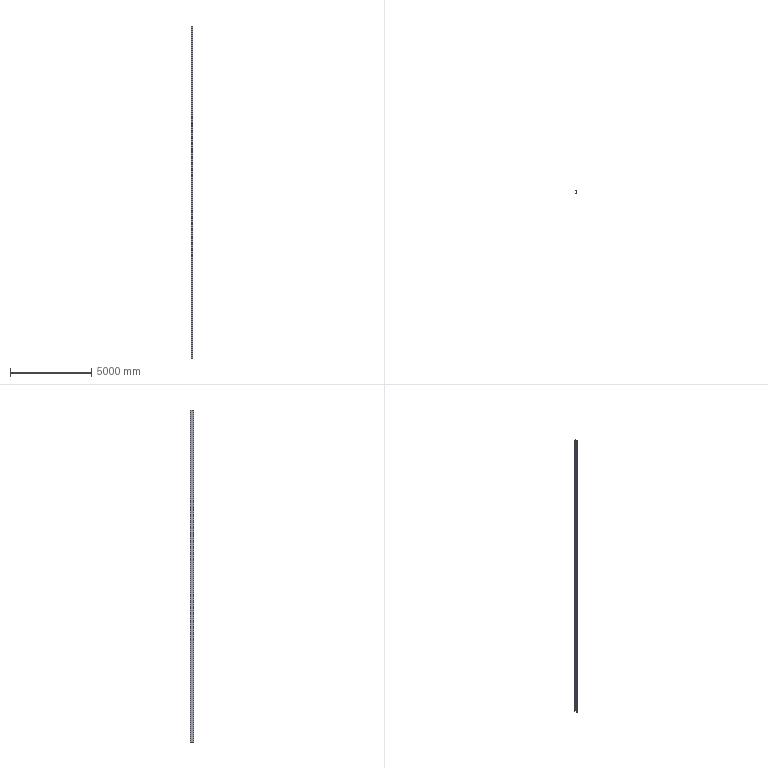Component | NX | P3 | 1 solid | 12 faces | box 73 x 200 x 20380 mm | volume 59182168 mm3 | plane 10 | cylinder 2 | commonest cylinder face diameters 22 x2
STEP:
#1=CARTESIAN_POINT('',(0.,0.,0.));
#2=DIRECTION('',(0.,0.,1.));
#3=DIRECTION('',(1.,0.,0.));
#4=AXIS2_PLACEMENT_3D('',#1,#2,#3);
#5=CARTESIAN_POINT('',(6830.,-6.,4.));
#6=VERTEX_POINT('',#5);
#7=CARTESIAN_POINT('',(6757.,-6.,4.));
#8=VERTEX_POINT('',#7);
#9=CARTESIAN_POINT('',(6830.,-6.,4.));
#10=DIRECTION('',(-1.,-0.,0.));
#11=VECTOR('',#10,1.);
#12=LINE('',#9,#11);
#13=CARTESIAN_POINT('',(6830.,-6.,20384.));
#14=DIRECTION('',(0.,-1.,0.));
#15=DIRECTION('',(-1.,-0.,0.));
#16=AXIS2_PLACEMENT_3D('',#13,#14,#15);
#17=PLANE('',#16);
#18=CARTESIAN_POINT('',(0.,20380.));
#19=DIRECTION('',(1.,0.));
#20=VECTOR('',#19,1.);
#21=LINE('',#18,#20);
#22=(GEOMETRIC_REPRESENTATION_CONTEXT(2)PARAMETRIC_REPRESENTATION_CONTEXT()REPRESENTATION_CONTEXT('',''));
#23=DEFINITIONAL_REPRESENTATION('',(#21),#22);
#24=PCURVE('',#17,#23);
#25=CARTESIAN_POINT('',(6812.,-28.,4.));
#26=DIRECTION('',(0.,0.,-1.));
#27=DIRECTION('',(0.,-1.,0.));
#28=AXIS2_PLACEMENT_3D('',#25,#26,#27);
#29=PLANE('',#28);
#30=CARTESIAN_POINT('',(-22.,-18.));
#31=DIRECTION('',(0.,1.));
#32=VECTOR('',#31,1.);
#33=LINE('',#30,#32);
#34=(GEOMETRIC_REPRESENTATION_CONTEXT(2)PARAMETRIC_REPRESENTATION_CONTEXT()REPRESENTATION_CONTEXT('',''));
#35=DEFINITIONAL_REPRESENTATION('',(#33),#34);
#36=PCURVE('',#29,#35);
#37=SURFACE_CURVE('',#12,(#24,#36),.PCURVE_S1.);
#38=EDGE_CURVE('',#6,#8,#37,.T.);
#39=ORIENTED_EDGE('',*,*,#38,.T.);
#40=CARTESIAN_POINT('',(6757.,-6.,20384.));
#41=VERTEX_POINT('',#40);
#42=CARTESIAN_POINT('',(6757.,-6.,20384.));
#43=DIRECTION('',(0.,0.,-1.));
#44=VECTOR('',#43,1.);
#45=LINE('',#42,#44);
#46=CARTESIAN_POINT('',(73.,0.));
#47=DIRECTION('',(0.,1.));
#48=VECTOR('',#47,1.);
#49=LINE('',#46,#48);
#50=(GEOMETRIC_REPRESENTATION_CONTEXT(2)PARAMETRIC_REPRESENTATION_CONTEXT()REPRESENTATION_CONTEXT('',''));
#51=DEFINITIONAL_REPRESENTATION('',(#49),#50);
#52=PCURVE('',#17,#51);
#53=CARTESIAN_POINT('',(6757.,-6.,20384.));
#54=DIRECTION('',(1.,0.,0.));
#55=DIRECTION('',(0.,0.,1.));
#56=AXIS2_PLACEMENT_3D('',#53,#54,#55);
#57=PLANE('',#56);
#58=CARTESIAN_POINT('',(0.,0.));
#59=DIRECTION('',(-1.,0.));
#60=VECTOR('',#59,1.);
#61=LINE('',#58,#60);
#62=(GEOMETRIC_REPRESENTATION_CONTEXT(2)PARAMETRIC_REPRESENTATION_CONTEXT()REPRESENTATION_CONTEXT('',''));
#63=DEFINITIONAL_REPRESENTATION('',(#61),#62);
#64=PCURVE('',#57,#63);
#65=SURFACE_CURVE('',#45,(#52,#64),.PCURVE_S1.);
#66=EDGE_CURVE('',#41,#8,#65,.T.);
#67=ORIENTED_EDGE('',*,*,#66,.F.);
#68=CARTESIAN_POINT('',(6830.,-6.,20384.));
#69=VERTEX_POINT('',#68);
#70=CARTESIAN_POINT('',(6830.,-6.,20384.));
#71=DIRECTION('',(-1.,-0.,0.));
#72=VECTOR('',#71,1.);
#73=LINE('',#70,#72);
#74=CARTESIAN_POINT('',(0.,0.));
#75=DIRECTION('',(1.,0.));
#76=VECTOR('',#75,1.);
#77=LINE('',#74,#76);
#78=(GEOMETRIC_REPRESENTATION_CONTEXT(2)PARAMETRIC_REPRESENTATION_CONTEXT()REPRESENTATION_CONTEXT('',''));
#79=DEFINITIONAL_REPRESENTATION('',(#77),#78);
#80=PCURVE('',#17,#79);
#81=CARTESIAN_POINT('',(6812.,-28.,20384.));
#82=DIRECTION('',(0.,0.,-1.));
#83=DIRECTION('',(0.,-1.,0.));
#84=AXIS2_PLACEMENT_3D('',#81,#82,#83);
#85=PLANE('',#84);
#86=CARTESIAN_POINT('',(-22.,-18.));
#87=DIRECTION('',(0.,1.));
#88=VECTOR('',#87,1.);
#89=LINE('',#86,#88);
#90=(GEOMETRIC_REPRESENTATION_CONTEXT(2)PARAMETRIC_REPRESENTATION_CONTEXT()REPRESENTATION_CONTEXT('',''));
#91=DEFINITIONAL_REPRESENTATION('',(#89),#90);
#92=PCURVE('',#85,#91);
#93=SURFACE_CURVE('',#73,(#80,#92),.PCURVE_S1.);
#94=EDGE_CURVE('',#69,#41,#93,.T.);
#95=ORIENTED_EDGE('',*,*,#94,.F.);
#96=CARTESIAN_POINT('',(6830.,-6.,20384.));
#97=DIRECTION('',(0.,0.,-1.));
#98=VECTOR('',#97,1.);
#99=LINE('',#96,#98);
#100=CARTESIAN_POINT('',(0.,0.));
#101=DIRECTION('',(0.,1.));
#102=VECTOR('',#101,1.);
#103=LINE('',#100,#102);
#104=(GEOMETRIC_REPRESENTATION_CONTEXT(2)PARAMETRIC_REPRESENTATION_CONTEXT()REPRESENTATION_CONTEXT('',''));
#105=DEFINITIONAL_REPRESENTATION('',(#103),#104);
#106=PCURVE('',#17,#105);
#107=CARTESIAN_POINT('',(6830.,-206.,20384.));
#108=DIRECTION('',(-1.,0.,0.));
#109=DIRECTION('',(0.,0.,-1.));
#110=AXIS2_PLACEMENT_3D('',#107,#108,#109);
#111=PLANE('',#110);
#112=CARTESIAN_POINT('',(0.,-200.));
#113=DIRECTION('',(1.,0.));
#114=VECTOR('',#113,1.);
#115=LINE('',#112,#114);
#116=(GEOMETRIC_REPRESENTATION_CONTEXT(2)PARAMETRIC_REPRESENTATION_CONTEXT()REPRESENTATION_CONTEXT('',''));
#117=DEFINITIONAL_REPRESENTATION('',(#115),#116);
#118=PCURVE('',#111,#117);
#119=SURFACE_CURVE('',#99,(#106,#118),.PCURVE_S1.);
#120=EDGE_CURVE('',#69,#6,#119,.T.);
#121=ORIENTED_EDGE('',*,*,#120,.T.);
#122=EDGE_LOOP('',(#39,#67,#95,#121));
#123=FACE_BOUND('',#122,.T.);
#124=ADVANCED_FACE('',(#123),#17,.F.);
#125=CARTESIAN_POINT('',(6757.,-17.,4.));
#126=VERTEX_POINT('',#125);
#127=CARTESIAN_POINT('',(6757.,-6.,4.));
#128=DIRECTION('',(0.,-1.,0.));
#129=VECTOR('',#128,1.);
#130=LINE('',#127,#129);
#131=CARTESIAN_POINT('',(-20380.,0.));
#132=DIRECTION('',(0.,1.));
#133=VECTOR('',#132,1.);
#134=LINE('',#131,#133);
#135=(GEOMETRIC_REPRESENTATION_CONTEXT(2)PARAMETRIC_REPRESENTATION_CONTEXT()REPRESENTATION_CONTEXT('',''));
#136=DEFINITIONAL_REPRESENTATION('',(#134),#135);
#137=PCURVE('',#57,#136);
#138=CARTESIAN_POINT('',(-22.,55.));
#139=DIRECTION('',(1.,0.));
#140=VECTOR('',#139,1.);
#141=LINE('',#138,#140);
#142=(GEOMETRIC_REPRESENTATION_CONTEXT(2)PARAMETRIC_REPRESENTATION_CONTEXT()REPRESENTATION_CONTEXT('',''));
#143=DEFINITIONAL_REPRESENTATION('',(#141),#142);
#144=PCURVE('',#29,#143);
#145=SURFACE_CURVE('',#130,(#137,#144),.PCURVE_S1.);
#146=EDGE_CURVE('',#8,#126,#145,.T.);
#147=ORIENTED_EDGE('',*,*,#146,.T.);
#148=CARTESIAN_POINT('',(6757.,-17.,20384.));
#149=VERTEX_POINT('',#148);
#150=CARTESIAN_POINT('',(6757.,-17.,20384.));
#151=DIRECTION('',(0.,0.,-1.));
#152=VECTOR('',#151,1.);
#153=LINE('',#150,#152);
#154=CARTESIAN_POINT('',(0.,11.));
#155=DIRECTION('',(-1.,0.));
#156=VECTOR('',#155,1.);
#157=LINE('',#154,#156);
#158=(GEOMETRIC_REPRESENTATION_CONTEXT(2)PARAMETRIC_REPRESENTATION_CONTEXT()REPRESENTATION_CONTEXT('',''));
#159=DEFINITIONAL_REPRESENTATION('',(#157),#158);
#160=PCURVE('',#57,#159);
#161=CARTESIAN_POINT('',(6757.,-17.,20384.));
#162=DIRECTION('',(-0.,1.,0.));
#163=DIRECTION('',(1.,0.,0.));
#164=AXIS2_PLACEMENT_3D('',#161,#162,#163);
#165=PLANE('',#164);
#166=CARTESIAN_POINT('',(0.,0.));
#167=DIRECTION('',(0.,1.));
#168=VECTOR('',#167,1.);
#169=LINE('',#166,#168);
#170=(GEOMETRIC_REPRESENTATION_CONTEXT(2)PARAMETRIC_REPRESENTATION_CONTEXT()REPRESENTATION_CONTEXT('',''));
#171=DEFINITIONAL_REPRESENTATION('',(#169),#170);
#172=PCURVE('',#165,#171);
#173=SURFACE_CURVE('',#153,(#160,#172),.PCURVE_S1.);
#174=EDGE_CURVE('',#149,#126,#173,.T.);
#175=ORIENTED_EDGE('',*,*,#174,.F.);
#176=CARTESIAN_POINT('',(6757.,-6.,20384.));
#177=DIRECTION('',(0.,-1.,0.));
#178=VECTOR('',#177,1.);
#179=LINE('',#176,#178);
#180=CARTESIAN_POINT('',(0.,0.));
#181=DIRECTION('',(0.,1.));
#182=VECTOR('',#181,1.);
#183=LINE('',#180,#182);
#184=(GEOMETRIC_REPRESENTATION_CONTEXT(2)PARAMETRIC_REPRESENTATION_CONTEXT()REPRESENTATION_CONTEXT('',''));
#185=DEFINITIONAL_REPRESENTATION('',(#183),#184);
#186=PCURVE('',#57,#185);
#187=CARTESIAN_POINT('',(-22.,55.));
#188=DIRECTION('',(1.,0.));
#189=VECTOR('',#188,1.);
#190=LINE('',#187,#189);
#191=(GEOMETRIC_REPRESENTATION_CONTEXT(2)PARAMETRIC_REPRESENTATION_CONTEXT()REPRESENTATION_CONTEXT('',''));
#192=DEFINITIONAL_REPRESENTATION('',(#190),#191);
#193=PCURVE('',#85,#192);
#194=SURFACE_CURVE('',#179,(#186,#193),.PCURVE_S1.);
#195=EDGE_CURVE('',#41,#149,#194,.T.);
#196=ORIENTED_EDGE('',*,*,#195,.F.);
#197=ORIENTED_EDGE('',*,*,#66,.T.);
#198=EDGE_LOOP('',(#147,#175,#196,#197));
#199=FACE_BOUND('',#198,.T.);
#200=ADVANCED_FACE('',(#199),#57,.F.);
#201=CARTESIAN_POINT('',(6812.,-17.,4.));
#202=VERTEX_POINT('',#201);
#203=CARTESIAN_POINT('',(6757.,-17.,4.));
#204=DIRECTION('',(1.,0.,0.));
#205=VECTOR('',#204,1.);
#206=LINE('',#203,#205);
#207=CARTESIAN_POINT('',(0.,20380.));
#208=DIRECTION('',(1.,0.));
#209=VECTOR('',#208,1.);
#210=LINE('',#207,#209);
#211=(GEOMETRIC_REPRESENTATION_CONTEXT(2)PARAMETRIC_REPRESENTATION_CONTEXT()REPRESENTATION_CONTEXT('',''));
#212=DEFINITIONAL_REPRESENTATION('',(#210),#211);
#213=PCURVE('',#165,#212);
#214=CARTESIAN_POINT('',(-11.,55.));
#215=DIRECTION('',(-0.,-1.));
#216=VECTOR('',#215,1.);
#217=LINE('',#214,#216);
#218=(GEOMETRIC_REPRESENTATION_CONTEXT(2)PARAMETRIC_REPRESENTATION_CONTEXT()REPRESENTATION_CONTEXT('',''));
#219=DEFINITIONAL_REPRESENTATION('',(#217),#218);
#220=PCURVE('',#29,#219);
#221=SURFACE_CURVE('',#206,(#213,#220),.PCURVE_S1.);
#222=EDGE_CURVE('',#126,#202,#221,.T.);
#223=ORIENTED_EDGE('',*,*,#222,.T.);
#224=CARTESIAN_POINT('',(6812.,-17.,20384.));
#225=VERTEX_POINT('',#224);
#226=CARTESIAN_POINT('',(6812.,-17.,20384.));
#227=DIRECTION('',(0.,0.,-1.));
#228=VECTOR('',#227,1.);
#229=LINE('',#226,#228);
#230=CARTESIAN_POINT('',(55.,0.));
#231=DIRECTION('',(0.,1.));
#232=VECTOR('',#231,1.);
#233=LINE('',#230,#232);
#234=(GEOMETRIC_REPRESENTATION_CONTEXT(2)PARAMETRIC_REPRESENTATION_CONTEXT()REPRESENTATION_CONTEXT('',''));
#235=DEFINITIONAL_REPRESENTATION('',(#233),#234);
#236=PCURVE('',#165,#235);
#237=CARTESIAN_POINT('',(6812.,-28.,20384.));
#238=DIRECTION('',(0.,0.,-1.));
#239=DIRECTION('',(0.,-1.,0.));
#240=AXIS2_PLACEMENT_3D('',#237,#238,#239);
#241=CYLINDRICAL_SURFACE('',#240,11.);
#242=CARTESIAN_POINT('',(3.142,0.));
#243=DIRECTION('',(0.,1.));
#244=VECTOR('',#243,1.);
#245=LINE('',#242,#244);
#246=(GEOMETRIC_REPRESENTATION_CONTEXT(2)PARAMETRIC_REPRESENTATION_CONTEXT()REPRESENTATION_CONTEXT('',''));
#247=DEFINITIONAL_REPRESENTATION('',(#245),#246);
#248=PCURVE('',#241,#247);
#249=SURFACE_CURVE('',#229,(#236,#248),.PCURVE_S1.);
#250=EDGE_CURVE('',#225,#202,#249,.T.);
#251=ORIENTED_EDGE('',*,*,#250,.F.);
#252=CARTESIAN_POINT('',(6757.,-17.,20384.));
#253=DIRECTION('',(1.,0.,0.));
#254=VECTOR('',#253,1.);
#255=LINE('',#252,#254);
#256=CARTESIAN_POINT('',(0.,0.));
#257=DIRECTION('',(1.,0.));
#258=VECTOR('',#257,1.);
#259=LINE('',#256,#258);
#260=(GEOMETRIC_REPRESENTATION_CONTEXT(2)PARAMETRIC_REPRESENTATION_CONTEXT()REPRESENTATION_CONTEXT('',''));
#261=DEFINITIONAL_REPRESENTATION('',(#259),#260);
#262=PCURVE('',#165,#261);
#263=CARTESIAN_POINT('',(-11.,55.));
#264=DIRECTION('',(-0.,-1.));
#265=VECTOR('',#264,1.);
#266=LINE('',#263,#265);
#267=(GEOMETRIC_REPRESENTATION_CONTEXT(2)PARAMETRIC_REPRESENTATION_CONTEXT()REPRESENTATION_CONTEXT('',''));
#268=DEFINITIONAL_REPRESENTATION('',(#266),#267);
#269=PCURVE('',#85,#268);
#270=SURFACE_CURVE('',#255,(#262,#269),.PCURVE_S1.);
#271=EDGE_CURVE('',#149,#225,#270,.T.);
#272=ORIENTED_EDGE('',*,*,#271,.F.);
#273=ORIENTED_EDGE('',*,*,#174,.T.);
#274=EDGE_LOOP('',(#223,#251,#272,#273));
#275=FACE_BOUND('',#274,.T.);
#276=ADVANCED_FACE('',(#275),#165,.F.);
#277=ORIENTED_EDGE('',*,*,#250,.F.);
#278=CARTESIAN_POINT('',(6823.,-28.,20384.));
#279=VERTEX_POINT('',#278);
#280=CARTESIAN_POINT('',(6812.,-28.,20384.));
#281=DIRECTION('',(0.,0.,-1.));
#282=DIRECTION('',(0.,-1.,0.));
#283=AXIS2_PLACEMENT_3D('',#280,#281,#282);
#284=CIRCLE('',#283,11.);
#285=CARTESIAN_POINT('',(0.,0.));
#286=DIRECTION('',(1.,0.));
#287=VECTOR('',#286,1.);
#288=LINE('',#285,#287);
#289=(GEOMETRIC_REPRESENTATION_CONTEXT(2)PARAMETRIC_REPRESENTATION_CONTEXT()REPRESENTATION_CONTEXT('',''));
#290=DEFINITIONAL_REPRESENTATION('',(#288),#289);
#291=PCURVE('',#241,#290);
#292=CARTESIAN_POINT('',(0.,0.));
#293=DIRECTION('',(1.,0.));
#294=AXIS2_PLACEMENT_2D('',#292,#293);
#295=CIRCLE('',#294,11.);
#296=(GEOMETRIC_REPRESENTATION_CONTEXT(2)PARAMETRIC_REPRESENTATION_CONTEXT()REPRESENTATION_CONTEXT('',''));
#297=DEFINITIONAL_REPRESENTATION('',(#295),#296);
#298=PCURVE('',#85,#297);
#299=SURFACE_CURVE('',#284,(#291,#298),.PCURVE_S1.);
#300=EDGE_CURVE('',#225,#279,#299,.T.);
#301=ORIENTED_EDGE('',*,*,#300,.T.);
#302=CARTESIAN_POINT('',(6823.,-28.,4.));
#303=VERTEX_POINT('',#302);
#304=CARTESIAN_POINT('',(6823.,-28.,20384.));
#305=DIRECTION('',(0.,0.,-1.));
#306=VECTOR('',#305,1.);
#307=LINE('',#304,#306);
#308=CARTESIAN_POINT('',(4.712,0.));
#309=DIRECTION('',(0.,1.));
#310=VECTOR('',#309,1.);
#311=LINE('',#308,#310);
#312=(GEOMETRIC_REPRESENTATION_CONTEXT(2)PARAMETRIC_REPRESENTATION_CONTEXT()REPRESENTATION_CONTEXT('',''));
#313=DEFINITIONAL_REPRESENTATION('',(#311),#312);
#314=PCURVE('',#241,#313);
#315=CARTESIAN_POINT('',(6823.,-28.,20384.));
#316=DIRECTION('',(1.,0.,0.));
#317=DIRECTION('',(0.,0.,1.));
#318=AXIS2_PLACEMENT_3D('',#315,#316,#317);
#319=PLANE('',#318);
#320=CARTESIAN_POINT('',(0.,0.));
#321=DIRECTION('',(-1.,0.));
#322=VECTOR('',#321,1.);
#323=LINE('',#320,#322);
#324=(GEOMETRIC_REPRESENTATION_CONTEXT(2)PARAMETRIC_REPRESENTATION_CONTEXT()REPRESENTATION_CONTEXT('',''));
#325=DEFINITIONAL_REPRESENTATION('',(#323),#324);
#326=PCURVE('',#319,#325);
#327=SURFACE_CURVE('',#307,(#314,#326),.PCURVE_S1.);
#328=EDGE_CURVE('',#279,#303,#327,.T.);
#329=ORIENTED_EDGE('',*,*,#328,.T.);
#330=CARTESIAN_POINT('',(6812.,-28.,4.));
#331=DIRECTION('',(0.,0.,-1.));
#332=DIRECTION('',(0.,-1.,0.));
#333=AXIS2_PLACEMENT_3D('',#330,#331,#332);
#334=CIRCLE('',#333,11.);
#335=CARTESIAN_POINT('',(0.,20380.));
#336=DIRECTION('',(1.,0.));
#337=VECTOR('',#336,1.);
#338=LINE('',#335,#337);
#339=(GEOMETRIC_REPRESENTATION_CONTEXT(2)PARAMETRIC_REPRESENTATION_CONTEXT()REPRESENTATION_CONTEXT('',''));
#340=DEFINITIONAL_REPRESENTATION('',(#338),#339);
#341=PCURVE('',#241,#340);
#342=CARTESIAN_POINT('',(0.,0.));
#343=DIRECTION('',(1.,0.));
#344=AXIS2_PLACEMENT_2D('',#342,#343);
#345=CIRCLE('',#344,11.);
#346=(GEOMETRIC_REPRESENTATION_CONTEXT(2)PARAMETRIC_REPRESENTATION_CONTEXT()REPRESENTATION_CONTEXT('',''));
#347=DEFINITIONAL_REPRESENTATION('',(#345),#346);
#348=PCURVE('',#29,#347);
#349=SURFACE_CURVE('',#334,(#341,#348),.PCURVE_S1.);
#350=EDGE_CURVE('',#202,#303,#349,.T.);
#351=ORIENTED_EDGE('',*,*,#350,.F.);
#352=EDGE_LOOP('',(#277,#301,#329,#351));
#353=FACE_BOUND('',#352,.F.);
#354=ADVANCED_FACE('',(#353),#241,.F.);
#355=CARTESIAN_POINT('',(6823.,-184.,4.));
#356=VERTEX_POINT('',#355);
#357=CARTESIAN_POINT('',(6823.,-28.,4.));
#358=DIRECTION('',(0.,-1.,0.));
#359=VECTOR('',#358,1.);
#360=LINE('',#357,#359);
#361=CARTESIAN_POINT('',(-20380.,0.));
#362=DIRECTION('',(0.,1.));
#363=VECTOR('',#362,1.);
#364=LINE('',#361,#363);
#365=(GEOMETRIC_REPRESENTATION_CONTEXT(2)PARAMETRIC_REPRESENTATION_CONTEXT()REPRESENTATION_CONTEXT('',''));
#366=DEFINITIONAL_REPRESENTATION('',(#364),#365);
#367=PCURVE('',#319,#366);
#368=CARTESIAN_POINT('',(0.,-11.));
#369=DIRECTION('',(1.,0.));
#370=VECTOR('',#369,1.);
#371=LINE('',#368,#370);
#372=(GEOMETRIC_REPRESENTATION_CONTEXT(2)PARAMETRIC_REPRESENTATION_CONTEXT()REPRESENTATION_CONTEXT('',''));
#373=DEFINITIONAL_REPRESENTATION('',(#371),#372);
#374=PCURVE('',#29,#373);
#375=SURFACE_CURVE('',#360,(#367,#374),.PCURVE_S1.);
#376=EDGE_CURVE('',#303,#356,#375,.T.);
#377=ORIENTED_EDGE('',*,*,#376,.T.);
#378=CARTESIAN_POINT('',(6823.,-184.,20384.));
#379=VERTEX_POINT('',#378);
#380=CARTESIAN_POINT('',(6823.,-184.,20384.));
#381=DIRECTION('',(0.,0.,-1.));
#382=VECTOR('',#381,1.);
#383=LINE('',#380,#382);
#384=CARTESIAN_POINT('',(0.,156.));
#385=DIRECTION('',(-1.,0.));
#386=VECTOR('',#385,1.);
#387=LINE('',#384,#386);
#388=(GEOMETRIC_REPRESENTATION_CONTEXT(2)PARAMETRIC_REPRESENTATION_CONTEXT()REPRESENTATION_CONTEXT('',''));
#389=DEFINITIONAL_REPRESENTATION('',(#387),#388);
#390=PCURVE('',#319,#389);
#391=CARTESIAN_POINT('',(6812.,-184.,20384.));
#392=DIRECTION('',(0.,0.,-1.));
#393=DIRECTION('',(0.,-1.,0.));
#394=AXIS2_PLACEMENT_3D('',#391,#392,#393);
#395=CYLINDRICAL_SURFACE('',#394,11.);
#396=CARTESIAN_POINT('',(4.712,0.));
#397=DIRECTION('',(0.,1.));
#398=VECTOR('',#397,1.);
#399=LINE('',#396,#398);
#400=(GEOMETRIC_REPRESENTATION_CONTEXT(2)PARAMETRIC_REPRESENTATION_CONTEXT()REPRESENTATION_CONTEXT('',''));
#401=DEFINITIONAL_REPRESENTATION('',(#399),#400);
#402=PCURVE('',#395,#401);
#403=SURFACE_CURVE('',#383,(#390,#402),.PCURVE_S1.);
#404=EDGE_CURVE('',#379,#356,#403,.T.);
#405=ORIENTED_EDGE('',*,*,#404,.F.);
#406=CARTESIAN_POINT('',(6823.,-28.,20384.));
#407=DIRECTION('',(0.,-1.,0.));
#408=VECTOR('',#407,1.);
#409=LINE('',#406,#408);
#410=CARTESIAN_POINT('',(0.,0.));
#411=DIRECTION('',(0.,1.));
#412=VECTOR('',#411,1.);
#413=LINE('',#410,#412);
#414=(GEOMETRIC_REPRESENTATION_CONTEXT(2)PARAMETRIC_REPRESENTATION_CONTEXT()REPRESENTATION_CONTEXT('',''));
#415=DEFINITIONAL_REPRESENTATION('',(#413),#414);
#416=PCURVE('',#319,#415);
#417=CARTESIAN_POINT('',(0.,-11.));
#418=DIRECTION('',(1.,0.));
#419=VECTOR('',#418,1.);
#420=LINE('',#417,#419);
#421=(GEOMETRIC_REPRESENTATION_CONTEXT(2)PARAMETRIC_REPRESENTATION_CONTEXT()REPRESENTATION_CONTEXT('',''));
#422=DEFINITIONAL_REPRESENTATION('',(#420),#421);
#423=PCURVE('',#85,#422);
#424=SURFACE_CURVE('',#409,(#416,#423),.PCURVE_S1.);
#425=EDGE_CURVE('',#279,#379,#424,.T.);
#426=ORIENTED_EDGE('',*,*,#425,.F.);
#427=ORIENTED_EDGE('',*,*,#328,.T.);
#428=EDGE_LOOP('',(#377,#405,#426,#427));
#429=FACE_BOUND('',#428,.T.);
#430=ADVANCED_FACE('',(#429),#319,.F.);
#431=ORIENTED_EDGE('',*,*,#404,.F.);
#432=CARTESIAN_POINT('',(6812.,-195.,20384.));
#433=VERTEX_POINT('',#432);
#434=CARTESIAN_POINT('',(6812.,-184.,20384.));
#435=DIRECTION('',(0.,0.,-1.));
#436=DIRECTION('',(0.,-1.,0.));
#437=AXIS2_PLACEMENT_3D('',#434,#435,#436);
#438=CIRCLE('',#437,11.);
#439=CARTESIAN_POINT('',(0.,0.));
#440=DIRECTION('',(1.,0.));
#441=VECTOR('',#440,1.);
#442=LINE('',#439,#441);
#443=(GEOMETRIC_REPRESENTATION_CONTEXT(2)PARAMETRIC_REPRESENTATION_CONTEXT()REPRESENTATION_CONTEXT('',''));
#444=DEFINITIONAL_REPRESENTATION('',(#442),#443);
#445=PCURVE('',#395,#444);
#446=CARTESIAN_POINT('',(156.,0.));
#447=DIRECTION('',(1.,0.));
#448=AXIS2_PLACEMENT_2D('',#446,#447);
#449=CIRCLE('',#448,11.);
#450=(GEOMETRIC_REPRESENTATION_CONTEXT(2)PARAMETRIC_REPRESENTATION_CONTEXT()REPRESENTATION_CONTEXT('',''));
#451=DEFINITIONAL_REPRESENTATION('',(#449),#450);
#452=PCURVE('',#85,#451);
#453=SURFACE_CURVE('',#438,(#445,#452),.PCURVE_S1.);
#454=EDGE_CURVE('',#379,#433,#453,.T.);
#455=ORIENTED_EDGE('',*,*,#454,.T.);
#456=CARTESIAN_POINT('',(6812.,-195.,4.));
#457=VERTEX_POINT('',#456);
#458=CARTESIAN_POINT('',(6812.,-195.,20384.));
#459=DIRECTION('',(0.,0.,-1.));
#460=VECTOR('',#459,1.);
#461=LINE('',#458,#460);
#462=CARTESIAN_POINT('',(6.283,0.));
#463=DIRECTION('',(0.,1.));
#464=VECTOR('',#463,1.);
#465=LINE('',#462,#464);
#466=(GEOMETRIC_REPRESENTATION_CONTEXT(2)PARAMETRIC_REPRESENTATION_CONTEXT()REPRESENTATION_CONTEXT('',''));
#467=DEFINITIONAL_REPRESENTATION('',(#465),#466);
#468=PCURVE('',#395,#467);
#469=CARTESIAN_POINT('',(6812.,-195.,20384.));
#470=DIRECTION('',(0.,-1.,0.));
#471=DIRECTION('',(-1.,-0.,0.));
#472=AXIS2_PLACEMENT_3D('',#469,#470,#471);
#473=PLANE('',#472);
#474=CARTESIAN_POINT('',(0.,0.));
#475=DIRECTION('',(0.,1.));
#476=VECTOR('',#475,1.);
#477=LINE('',#474,#476);
#478=(GEOMETRIC_REPRESENTATION_CONTEXT(2)PARAMETRIC_REPRESENTATION_CONTEXT()REPRESENTATION_CONTEXT('',''));
#479=DEFINITIONAL_REPRESENTATION('',(#477),#478);
#480=PCURVE('',#473,#479);
#481=SURFACE_CURVE('',#461,(#468,#480),.PCURVE_S1.);
#482=EDGE_CURVE('',#433,#457,#481,.T.);
#483=ORIENTED_EDGE('',*,*,#482,.T.);
#484=CARTESIAN_POINT('',(6812.,-184.,4.));
#485=DIRECTION('',(0.,0.,-1.));
#486=DIRECTION('',(0.,-1.,0.));
#487=AXIS2_PLACEMENT_3D('',#484,#485,#486);
#488=CIRCLE('',#487,11.);
#489=CARTESIAN_POINT('',(0.,20380.));
#490=DIRECTION('',(1.,0.));
#491=VECTOR('',#490,1.);
#492=LINE('',#489,#491);
#493=(GEOMETRIC_REPRESENTATION_CONTEXT(2)PARAMETRIC_REPRESENTATION_CONTEXT()REPRESENTATION_CONTEXT('',''));
#494=DEFINITIONAL_REPRESENTATION('',(#492),#493);
#495=PCURVE('',#395,#494);
#496=CARTESIAN_POINT('',(156.,0.));
#497=DIRECTION('',(1.,0.));
#498=AXIS2_PLACEMENT_2D('',#496,#497);
#499=CIRCLE('',#498,11.);
#500=(GEOMETRIC_REPRESENTATION_CONTEXT(2)PARAMETRIC_REPRESENTATION_CONTEXT()REPRESENTATION_CONTEXT('',''));
#501=DEFINITIONAL_REPRESENTATION('',(#499),#500);
#502=PCURVE('',#29,#501);
#503=SURFACE_CURVE('',#488,(#495,#502),.PCURVE_S1.);
#504=EDGE_CURVE('',#356,#457,#503,.T.);
#505=ORIENTED_EDGE('',*,*,#504,.F.);
#506=EDGE_LOOP('',(#431,#455,#483,#505));
#507=FACE_BOUND('',#506,.F.);
#508=ADVANCED_FACE('',(#507),#395,.F.);
#509=CARTESIAN_POINT('',(6757.,-195.,4.));
#510=VERTEX_POINT('',#509);
#511=CARTESIAN_POINT('',(6812.,-195.,4.));
#512=DIRECTION('',(-1.,-0.,0.));
#513=VECTOR('',#512,1.);
#514=LINE('',#511,#513);
#515=CARTESIAN_POINT('',(0.,20380.));
#516=DIRECTION('',(1.,0.));
#517=VECTOR('',#516,1.);
#518=LINE('',#515,#517);
#519=(GEOMETRIC_REPRESENTATION_CONTEXT(2)PARAMETRIC_REPRESENTATION_CONTEXT()REPRESENTATION_CONTEXT('',''));
#520=DEFINITIONAL_REPRESENTATION('',(#518),#519);
#521=PCURVE('',#473,#520);
#522=CARTESIAN_POINT('',(167.,0.));
#523=DIRECTION('',(0.,1.));
#524=VECTOR('',#523,1.);
#525=LINE('',#522,#524);
#526=(GEOMETRIC_REPRESENTATION_CONTEXT(2)PARAMETRIC_REPRESENTATION_CONTEXT()REPRESENTATION_CONTEXT('',''));
#527=DEFINITIONAL_REPRESENTATION('',(#525),#526);
#528=PCURVE('',#29,#527);
#529=SURFACE_CURVE('',#514,(#521,#528),.PCURVE_S1.);
#530=EDGE_CURVE('',#457,#510,#529,.T.);
#531=ORIENTED_EDGE('',*,*,#530,.T.);
#532=CARTESIAN_POINT('',(6757.,-195.,20384.));
#533=VERTEX_POINT('',#532);
#534=CARTESIAN_POINT('',(6757.,-195.,20384.));
#535=DIRECTION('',(0.,0.,-1.));
#536=VECTOR('',#535,1.);
#537=LINE('',#534,#536);
#538=CARTESIAN_POINT('',(55.,0.));
#539=DIRECTION('',(0.,1.));
#540=VECTOR('',#539,1.);
#541=LINE('',#538,#540);
#542=(GEOMETRIC_REPRESENTATION_CONTEXT(2)PARAMETRIC_REPRESENTATION_CONTEXT()REPRESENTATION_CONTEXT('',''));
#543=DEFINITIONAL_REPRESENTATION('',(#541),#542);
#544=PCURVE('',#473,#543);
#545=CARTESIAN_POINT('',(6757.,-195.,20384.));
#546=DIRECTION('',(1.,0.,0.));
#547=DIRECTION('',(0.,0.,1.));
#548=AXIS2_PLACEMENT_3D('',#545,#546,#547);
#549=PLANE('',#548);
#550=CARTESIAN_POINT('',(0.,0.));
#551=DIRECTION('',(-1.,0.));
#552=VECTOR('',#551,1.);
#553=LINE('',#550,#552);
#554=(GEOMETRIC_REPRESENTATION_CONTEXT(2)PARAMETRIC_REPRESENTATION_CONTEXT()REPRESENTATION_CONTEXT('',''));
#555=DEFINITIONAL_REPRESENTATION('',(#553),#554);
#556=PCURVE('',#549,#555);
#557=SURFACE_CURVE('',#537,(#544,#556),.PCURVE_S1.);
#558=EDGE_CURVE('',#533,#510,#557,.T.);
#559=ORIENTED_EDGE('',*,*,#558,.F.);
#560=CARTESIAN_POINT('',(6812.,-195.,20384.));
#561=DIRECTION('',(-1.,-0.,0.));
#562=VECTOR('',#561,1.);
#563=LINE('',#560,#562);
#564=CARTESIAN_POINT('',(0.,0.));
#565=DIRECTION('',(1.,0.));
#566=VECTOR('',#565,1.);
#567=LINE('',#564,#566);
#568=(GEOMETRIC_REPRESENTATION_CONTEXT(2)PARAMETRIC_REPRESENTATION_CONTEXT()REPRESENTATION_CONTEXT('',''));
#569=DEFINITIONAL_REPRESENTATION('',(#567),#568);
#570=PCURVE('',#473,#569);
#571=CARTESIAN_POINT('',(167.,0.));
#572=DIRECTION('',(0.,1.));
#573=VECTOR('',#572,1.);
#574=LINE('',#571,#573);
#575=(GEOMETRIC_REPRESENTATION_CONTEXT(2)PARAMETRIC_REPRESENTATION_CONTEXT()REPRESENTATION_CONTEXT('',''));
#576=DEFINITIONAL_REPRESENTATION('',(#574),#575);
#577=PCURVE('',#85,#576);
#578=SURFACE_CURVE('',#563,(#570,#577),.PCURVE_S1.);
#579=EDGE_CURVE('',#433,#533,#578,.T.);
#580=ORIENTED_EDGE('',*,*,#579,.F.);
#581=ORIENTED_EDGE('',*,*,#482,.T.);
#582=EDGE_LOOP('',(#531,#559,#580,#581));
#583=FACE_BOUND('',#582,.T.);
#584=ADVANCED_FACE('',(#583),#473,.F.);
#585=CARTESIAN_POINT('',(6757.,-206.,4.));
#586=VERTEX_POINT('',#585);
#587=CARTESIAN_POINT('',(6757.,-195.,4.));
#588=DIRECTION('',(0.,-1.,0.));
#589=VECTOR('',#588,1.);
#590=LINE('',#587,#589);
#591=CARTESIAN_POINT('',(-20380.,0.));
#592=DIRECTION('',(0.,1.));
#593=VECTOR('',#592,1.);
#594=LINE('',#591,#593);
#595=(GEOMETRIC_REPRESENTATION_CONTEXT(2)PARAMETRIC_REPRESENTATION_CONTEXT()REPRESENTATION_CONTEXT('',''));
#596=DEFINITIONAL_REPRESENTATION('',(#594),#595);
#597=PCURVE('',#549,#596);
#598=CARTESIAN_POINT('',(167.,55.));
#599=DIRECTION('',(1.,0.));
#600=VECTOR('',#599,1.);
#601=LINE('',#598,#600);
#602=(GEOMETRIC_REPRESENTATION_CONTEXT(2)PARAMETRIC_REPRESENTATION_CONTEXT()REPRESENTATION_CONTEXT('',''));
#603=DEFINITIONAL_REPRESENTATION('',(#601),#602);
#604=PCURVE('',#29,#603);
#605=SURFACE_CURVE('',#590,(#597,#604),.PCURVE_S1.);
#606=EDGE_CURVE('',#510,#586,#605,.T.);
#607=ORIENTED_EDGE('',*,*,#606,.T.);
#608=CARTESIAN_POINT('',(6757.,-206.,20384.));
#609=VERTEX_POINT('',#608);
#610=CARTESIAN_POINT('',(6757.,-206.,20384.));
#611=DIRECTION('',(0.,0.,-1.));
#612=VECTOR('',#611,1.);
#613=LINE('',#610,#612);
#614=CARTESIAN_POINT('',(0.,11.));
#615=DIRECTION('',(-1.,0.));
#616=VECTOR('',#615,1.);
#617=LINE('',#614,#616);
#618=(GEOMETRIC_REPRESENTATION_CONTEXT(2)PARAMETRIC_REPRESENTATION_CONTEXT()REPRESENTATION_CONTEXT('',''));
#619=DEFINITIONAL_REPRESENTATION('',(#617),#618);
#620=PCURVE('',#549,#619);
#621=CARTESIAN_POINT('',(6757.,-206.,20384.));
#622=DIRECTION('',(-0.,1.,0.));
#623=DIRECTION('',(1.,0.,0.));
#624=AXIS2_PLACEMENT_3D('',#621,#622,#623);
#625=PLANE('',#624);
#626=CARTESIAN_POINT('',(0.,0.));
#627=DIRECTION('',(0.,1.));
#628=VECTOR('',#627,1.);
#629=LINE('',#626,#628);
#630=(GEOMETRIC_REPRESENTATION_CONTEXT(2)PARAMETRIC_REPRESENTATION_CONTEXT()REPRESENTATION_CONTEXT('',''));
#631=DEFINITIONAL_REPRESENTATION('',(#629),#630);
#632=PCURVE('',#625,#631);
#633=SURFACE_CURVE('',#613,(#620,#632),.PCURVE_S1.);
#634=EDGE_CURVE('',#609,#586,#633,.T.);
#635=ORIENTED_EDGE('',*,*,#634,.F.);
#636=CARTESIAN_POINT('',(6757.,-195.,20384.));
#637=DIRECTION('',(0.,-1.,0.));
#638=VECTOR('',#637,1.);
#639=LINE('',#636,#638);
#640=CARTESIAN_POINT('',(0.,0.));
#641=DIRECTION('',(0.,1.));
#642=VECTOR('',#641,1.);
#643=LINE('',#640,#642);
#644=(GEOMETRIC_REPRESENTATION_CONTEXT(2)PARAMETRIC_REPRESENTATION_CONTEXT()REPRESENTATION_CONTEXT('',''));
#645=DEFINITIONAL_REPRESENTATION('',(#643),#644);
#646=PCURVE('',#549,#645);
#647=CARTESIAN_POINT('',(167.,55.));
#648=DIRECTION('',(1.,0.));
#649=VECTOR('',#648,1.);
#650=LINE('',#647,#649);
#651=(GEOMETRIC_REPRESENTATION_CONTEXT(2)PARAMETRIC_REPRESENTATION_CONTEXT()REPRESENTATION_CONTEXT('',''));
#652=DEFINITIONAL_REPRESENTATION('',(#650),#651);
#653=PCURVE('',#85,#652);
#654=SURFACE_CURVE('',#639,(#646,#653),.PCURVE_S1.);
#655=EDGE_CURVE('',#533,#609,#654,.T.);
#656=ORIENTED_EDGE('',*,*,#655,.F.);
#657=ORIENTED_EDGE('',*,*,#558,.T.);
#658=EDGE_LOOP('',(#607,#635,#656,#657));
#659=FACE_BOUND('',#658,.T.);
#660=ADVANCED_FACE('',(#659),#549,.F.);
#661=CARTESIAN_POINT('',(6830.,-206.,4.));
#662=VERTEX_POINT('',#661);
#663=CARTESIAN_POINT('',(6757.,-206.,4.));
#664=DIRECTION('',(1.,0.,0.));
#665=VECTOR('',#664,1.);
#666=LINE('',#663,#665);
#667=CARTESIAN_POINT('',(0.,20380.));
#668=DIRECTION('',(1.,0.));
#669=VECTOR('',#668,1.);
#670=LINE('',#667,#669);
#671=(GEOMETRIC_REPRESENTATION_CONTEXT(2)PARAMETRIC_REPRESENTATION_CONTEXT()REPRESENTATION_CONTEXT('',''));
#672=DEFINITIONAL_REPRESENTATION('',(#670),#671);
#673=PCURVE('',#625,#672);
#674=CARTESIAN_POINT('',(178.,55.));
#675=DIRECTION('',(-0.,-1.));
#676=VECTOR('',#675,1.);
#677=LINE('',#674,#676);
#678=(GEOMETRIC_REPRESENTATION_CONTEXT(2)PARAMETRIC_REPRESENTATION_CONTEXT()REPRESENTATION_CONTEXT('',''));
#679=DEFINITIONAL_REPRESENTATION('',(#677),#678);
#680=PCURVE('',#29,#679);
#681=SURFACE_CURVE('',#666,(#673,#680),.PCURVE_S1.);
#682=EDGE_CURVE('',#586,#662,#681,.T.);
#683=ORIENTED_EDGE('',*,*,#682,.T.);
#684=CARTESIAN_POINT('',(6830.,-206.,20384.));
#685=VERTEX_POINT('',#684);
#686=CARTESIAN_POINT('',(6830.,-206.,20384.));
#687=DIRECTION('',(0.,0.,-1.));
#688=VECTOR('',#687,1.);
#689=LINE('',#686,#688);
#690=CARTESIAN_POINT('',(73.,0.));
#691=DIRECTION('',(0.,1.));
#692=VECTOR('',#691,1.);
#693=LINE('',#690,#692);
#694=(GEOMETRIC_REPRESENTATION_CONTEXT(2)PARAMETRIC_REPRESENTATION_CONTEXT()REPRESENTATION_CONTEXT('',''));
#695=DEFINITIONAL_REPRESENTATION('',(#693),#694);
#696=PCURVE('',#625,#695);
#697=CARTESIAN_POINT('',(0.,0.));
#698=DIRECTION('',(1.,0.));
#699=VECTOR('',#698,1.);
#700=LINE('',#697,#699);
#701=(GEOMETRIC_REPRESENTATION_CONTEXT(2)PARAMETRIC_REPRESENTATION_CONTEXT()REPRESENTATION_CONTEXT('',''));
#702=DEFINITIONAL_REPRESENTATION('',(#700),#701);
#703=PCURVE('',#111,#702);
#704=SURFACE_CURVE('',#689,(#696,#703),.PCURVE_S1.);
#705=EDGE_CURVE('',#685,#662,#704,.T.);
#706=ORIENTED_EDGE('',*,*,#705,.F.);
#707=CARTESIAN_POINT('',(6757.,-206.,20384.));
#708=DIRECTION('',(1.,0.,0.));
#709=VECTOR('',#708,1.);
#710=LINE('',#707,#709);
#711=CARTESIAN_POINT('',(0.,0.));
#712=DIRECTION('',(1.,0.));
#713=VECTOR('',#712,1.);
#714=LINE('',#711,#713);
#715=(GEOMETRIC_REPRESENTATION_CONTEXT(2)PARAMETRIC_REPRESENTATION_CONTEXT()REPRESENTATION_CONTEXT('',''));
#716=DEFINITIONAL_REPRESENTATION('',(#714),#715);
#717=PCURVE('',#625,#716);
#718=CARTESIAN_POINT('',(178.,55.));
#719=DIRECTION('',(-0.,-1.));
#720=VECTOR('',#719,1.);
#721=LINE('',#718,#720);
#722=(GEOMETRIC_REPRESENTATION_CONTEXT(2)PARAMETRIC_REPRESENTATION_CONTEXT()REPRESENTATION_CONTEXT('',''));
#723=DEFINITIONAL_REPRESENTATION('',(#721),#722);
#724=PCURVE('',#85,#723);
#725=SURFACE_CURVE('',#710,(#717,#724),.PCURVE_S1.);
#726=EDGE_CURVE('',#609,#685,#725,.T.);
#727=ORIENTED_EDGE('',*,*,#726,.F.);
#728=ORIENTED_EDGE('',*,*,#634,.T.);
#729=EDGE_LOOP('',(#683,#706,#727,#728));
#730=FACE_BOUND('',#729,.T.);
#731=ADVANCED_FACE('',(#730),#625,.F.);
#732=CARTESIAN_POINT('',(6830.,-206.,4.));
#733=DIRECTION('',(0.,1.,0.));
#734=VECTOR('',#733,1.);
#735=LINE('',#732,#734);
#736=CARTESIAN_POINT('',(20380.,0.));
#737=DIRECTION('',(0.,-1.));
#738=VECTOR('',#737,1.);
#739=LINE('',#736,#738);
#740=(GEOMETRIC_REPRESENTATION_CONTEXT(2)PARAMETRIC_REPRESENTATION_CONTEXT()REPRESENTATION_CONTEXT('',''));
#741=DEFINITIONAL_REPRESENTATION('',(#739),#740);
#742=PCURVE('',#111,#741);
#743=CARTESIAN_POINT('',(178.,-18.));
#744=DIRECTION('',(-1.,0.));
#745=VECTOR('',#744,1.);
#746=LINE('',#743,#745);
#747=(GEOMETRIC_REPRESENTATION_CONTEXT(2)PARAMETRIC_REPRESENTATION_CONTEXT()REPRESENTATION_CONTEXT('',''));
#748=DEFINITIONAL_REPRESENTATION('',(#746),#747);
#749=PCURVE('',#29,#748);
#750=SURFACE_CURVE('',#735,(#742,#749),.PCURVE_S1.);
#751=EDGE_CURVE('',#662,#6,#750,.T.);
#752=ORIENTED_EDGE('',*,*,#751,.T.);
#753=ORIENTED_EDGE('',*,*,#120,.F.);
#754=CARTESIAN_POINT('',(6830.,-206.,20384.));
#755=DIRECTION('',(0.,1.,0.));
#756=VECTOR('',#755,1.);
#757=LINE('',#754,#756);
#758=CARTESIAN_POINT('',(0.,0.));
#759=DIRECTION('',(0.,-1.));
#760=VECTOR('',#759,1.);
#761=LINE('',#758,#760);
#762=(GEOMETRIC_REPRESENTATION_CONTEXT(2)PARAMETRIC_REPRESENTATION_CONTEXT()REPRESENTATION_CONTEXT('',''));
#763=DEFINITIONAL_REPRESENTATION('',(#761),#762);
#764=PCURVE('',#111,#763);
#765=CARTESIAN_POINT('',(178.,-18.));
#766=DIRECTION('',(-1.,0.));
#767=VECTOR('',#766,1.);
#768=LINE('',#765,#767);
#769=(GEOMETRIC_REPRESENTATION_CONTEXT(2)PARAMETRIC_REPRESENTATION_CONTEXT()REPRESENTATION_CONTEXT('',''));
#770=DEFINITIONAL_REPRESENTATION('',(#768),#769);
#771=PCURVE('',#85,#770);
#772=SURFACE_CURVE('',#757,(#764,#771),.PCURVE_S1.);
#773=EDGE_CURVE('',#685,#69,#772,.T.);
#774=ORIENTED_EDGE('',*,*,#773,.F.);
#775=ORIENTED_EDGE('',*,*,#705,.T.);
#776=EDGE_LOOP('',(#752,#753,#774,#775));
#777=FACE_BOUND('',#776,.T.);
#778=ADVANCED_FACE('',(#777),#111,.F.);
#779=ORIENTED_EDGE('',*,*,#94,.T.);
#780=ORIENTED_EDGE('',*,*,#195,.T.);
#781=ORIENTED_EDGE('',*,*,#271,.T.);
#782=ORIENTED_EDGE('',*,*,#300,.T.);
#783=ORIENTED_EDGE('',*,*,#425,.T.);
#784=ORIENTED_EDGE('',*,*,#454,.T.);
#785=ORIENTED_EDGE('',*,*,#579,.T.);
#786=ORIENTED_EDGE('',*,*,#655,.T.);
#787=ORIENTED_EDGE('',*,*,#726,.T.);
#788=ORIENTED_EDGE('',*,*,#773,.T.);
#789=EDGE_LOOP('',(#779,#780,#781,#782,#783,#784,#785,#786,#787,#788));
#790=FACE_BOUND('',#789,.T.);
#791=ADVANCED_FACE('',(#790),#85,.F.);
#792=ORIENTED_EDGE('',*,*,#38,.F.);
#793=ORIENTED_EDGE('',*,*,#751,.F.);
#794=ORIENTED_EDGE('',*,*,#682,.F.);
#795=ORIENTED_EDGE('',*,*,#606,.F.);
#796=ORIENTED_EDGE('',*,*,#530,.F.);
#797=ORIENTED_EDGE('',*,*,#504,.F.);
#798=ORIENTED_EDGE('',*,*,#376,.F.);
#799=ORIENTED_EDGE('',*,*,#350,.F.);
#800=ORIENTED_EDGE('',*,*,#222,.F.);
#801=ORIENTED_EDGE('',*,*,#146,.F.);
#802=EDGE_LOOP('',(#792,#793,#794,#795,#796,#797,#798,#799,#800,#801));
#803=FACE_BOUND('',#802,.T.);
#804=ADVANCED_FACE('',(#803),#29,.T.);
#805=CLOSED_SHELL('',(#124,#200,#276,#354,#430,#508,#584,#660,#731,#778,#791,#804));
#806=MANIFOLD_SOLID_BREP('',#805);
#807=(LENGTH_UNIT()NAMED_UNIT(*)SI_UNIT(.MILLI.,.METRE.));
#808=UNCERTAINTY_MEASURE_WITH_UNIT(LENGTH_MEASURE(0.0000001),#807,'','');
#809=(NAMED_UNIT(*)PLANE_ANGLE_UNIT()SI_UNIT($,.RADIAN.));
#810=(NAMED_UNIT(*)SI_UNIT($,.STERADIAN.)SOLID_ANGLE_UNIT());
#811=(GEOMETRIC_REPRESENTATION_CONTEXT(3)GLOBAL_UNCERTAINTY_ASSIGNED_CONTEXT((#808))GLOBAL_UNIT_ASSIGNED_CONTEXT((#807,#809,#810))REPRESENTATION_CONTEXT('',''));
#812=ADVANCED_BREP_SHAPE_REPRESENTATION('',(#4,#806),#811);